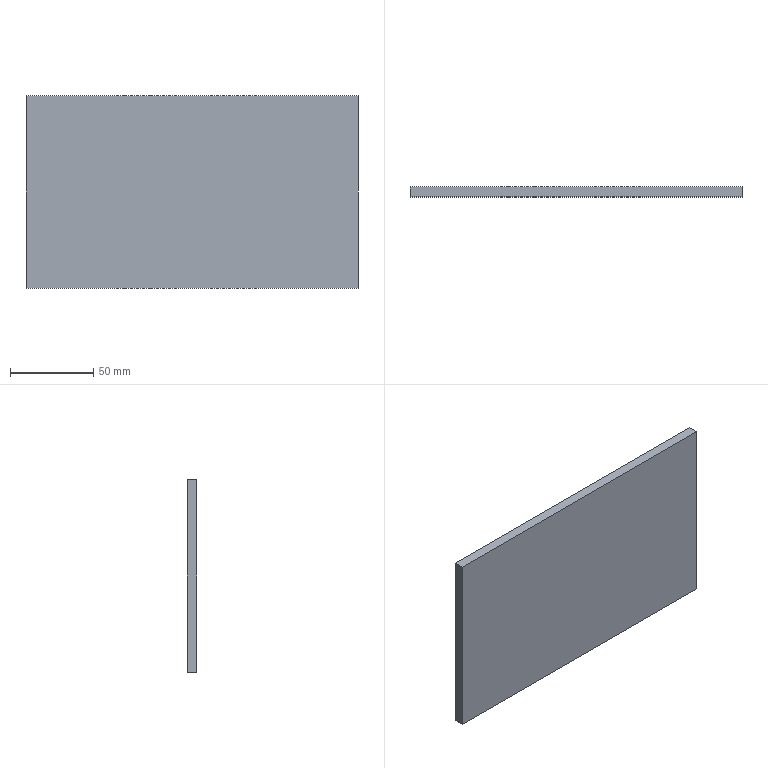Component | SolidWorks | THK-B1013LowerSupportPlate-4 | 1 solid | 6 faces | box 200 x 6 x 116 mm | volume 139200 mm3 | plane 6 | material Q235A
build123d program:
from build123d import *

# Parameters (mm, degrees)
SKETCH1_W           = 200
SKETCH1_H           = 116
BOSS_EXTRUDE1_DEPTH = 3


with BuildPart() as part:
    # Sketch1 → Boss-Extrude1 (new, symmetric)
    with BuildSketch(Plane(origin=(0, 0, 0), x_dir=(1, 0, 0), z_dir=(0, 1, 0))):
        Rectangle(SKETCH1_W, SKETCH1_H)
    extrude(amount=BOSS_EXTRUDE1_DEPTH, both=True)


solid = part.part

# Placed as in the assembly
solid = solid.moved(Location((222, -203, -200), (0, 0, 0)))
STEP:
#1=COLOUR_RGB('',0.7922,0.8196,0.9333);
#2=FILL_AREA_STYLE_COLOUR('',#1);
#3=FILL_AREA_STYLE('',(#2));
#4=SURFACE_STYLE_FILL_AREA(#3);
#5=SURFACE_SIDE_STYLE('',(#4));
#6=SURFACE_STYLE_USAGE(.BOTH.,#5);
#7=PRESENTATION_STYLE_ASSIGNMENT((#6));
#8=CARTESIAN_POINT('',(12.677,-8.11,-5.591));
#9=VERTEX_POINT('',#8);
#10=CARTESIAN_POINT('',(12.677,-8.11,-10.157));
#11=VERTEX_POINT('',#10);
#12=CARTESIAN_POINT('',(12.677,-8.11,-5.591));
#13=DIRECTION('',(0.,0.,-1.));
#14=VECTOR('',#13,39.37);
#15=LINE('',#12,#14);
#16=EDGE_CURVE('',#9,#11,#15,.T.);
#17=ORIENTED_EDGE('',*,*,#16,.T.);
#18=CARTESIAN_POINT('',(12.677,-7.874,-10.157));
#19=VERTEX_POINT('',#18);
#20=CARTESIAN_POINT('',(12.677,-7.874,-10.157));
#21=DIRECTION('',(0.,-1.,0.));
#22=VECTOR('',#21,39.37);
#23=LINE('',#20,#22);
#24=EDGE_CURVE('',#19,#11,#23,.T.);
#25=ORIENTED_EDGE('',*,*,#24,.F.);
#26=CARTESIAN_POINT('',(12.677,-7.874,-5.591));
#27=VERTEX_POINT('',#26);
#28=CARTESIAN_POINT('',(12.677,-7.874,-5.591));
#29=DIRECTION('',(0.,0.,-1.));
#30=VECTOR('',#29,39.37);
#31=LINE('',#28,#30);
#32=EDGE_CURVE('',#27,#19,#31,.T.);
#33=ORIENTED_EDGE('',*,*,#32,.F.);
#34=CARTESIAN_POINT('',(12.677,-7.874,-5.591));
#35=DIRECTION('',(0.,-1.,0.));
#36=VECTOR('',#35,39.37);
#37=LINE('',#34,#36);
#38=EDGE_CURVE('',#27,#9,#37,.T.);
#39=ORIENTED_EDGE('',*,*,#38,.T.);
#40=EDGE_LOOP('',(#17,#25,#33,#39));
#41=FACE_OUTER_BOUND('',#40,.T.);
#42=CARTESIAN_POINT('',(12.677,-7.874,-5.591));
#43=DIRECTION('',(-1.,0.,0.));
#44=DIRECTION('',(0.,0.,1.));
#45=AXIS2_PLACEMENT_3D('',#42,#43,#44);
#46=PLANE('',#45);
#47=ADVANCED_FACE('',(#41),#46,.F.);
#48=CARTESIAN_POINT('',(4.803,-8.11,-10.157));
#49=VERTEX_POINT('',#48);
#50=CARTESIAN_POINT('',(4.803,-8.11,-10.157));
#51=DIRECTION('',(-1.,0.,0.));
#52=VECTOR('',#51,39.37);
#53=LINE('',#50,#52);
#54=EDGE_CURVE('',#11,#49,#53,.T.);
#55=ORIENTED_EDGE('',*,*,#54,.T.);
#56=CARTESIAN_POINT('',(4.803,-7.874,-10.157));
#57=VERTEX_POINT('',#56);
#58=CARTESIAN_POINT('',(4.803,-7.874,-10.157));
#59=DIRECTION('',(0.,-1.,0.));
#60=VECTOR('',#59,39.37);
#61=LINE('',#58,#60);
#62=EDGE_CURVE('',#57,#49,#61,.T.);
#63=ORIENTED_EDGE('',*,*,#62,.F.);
#64=CARTESIAN_POINT('',(4.803,-7.874,-10.157));
#65=DIRECTION('',(-1.,0.,0.));
#66=VECTOR('',#65,39.37);
#67=LINE('',#64,#66);
#68=EDGE_CURVE('',#19,#57,#67,.T.);
#69=ORIENTED_EDGE('',*,*,#68,.F.);
#70=ORIENTED_EDGE('',*,*,#24,.T.);
#71=EDGE_LOOP('',(#55,#63,#69,#70));
#72=FACE_OUTER_BOUND('',#71,.T.);
#73=CARTESIAN_POINT('',(4.803,-7.874,-10.157));
#74=DIRECTION('',(0.,0.,1.));
#75=DIRECTION('',(1.,0.,0.));
#76=AXIS2_PLACEMENT_3D('',#73,#74,#75);
#77=PLANE('',#76);
#78=ADVANCED_FACE('',(#72),#77,.F.);
#79=CARTESIAN_POINT('',(4.803,-8.11,-5.591));
#80=VERTEX_POINT('',#79);
#81=CARTESIAN_POINT('',(4.803,-8.11,-5.591));
#82=DIRECTION('',(0.,0.,1.));
#83=VECTOR('',#82,39.37);
#84=LINE('',#81,#83);
#85=EDGE_CURVE('',#49,#80,#84,.T.);
#86=ORIENTED_EDGE('',*,*,#85,.T.);
#87=CARTESIAN_POINT('',(4.803,-7.874,-5.591));
#88=VERTEX_POINT('',#87);
#89=CARTESIAN_POINT('',(4.803,-7.874,-5.591));
#90=DIRECTION('',(0.,-1.,0.));
#91=VECTOR('',#90,39.37);
#92=LINE('',#89,#91);
#93=EDGE_CURVE('',#88,#80,#92,.T.);
#94=ORIENTED_EDGE('',*,*,#93,.F.);
#95=CARTESIAN_POINT('',(4.803,-7.874,-5.591));
#96=DIRECTION('',(0.,0.,1.));
#97=VECTOR('',#96,39.37);
#98=LINE('',#95,#97);
#99=EDGE_CURVE('',#57,#88,#98,.T.);
#100=ORIENTED_EDGE('',*,*,#99,.F.);
#101=ORIENTED_EDGE('',*,*,#62,.T.);
#102=EDGE_LOOP('',(#86,#94,#100,#101));
#103=FACE_OUTER_BOUND('',#102,.T.);
#104=CARTESIAN_POINT('',(4.803,-7.874,-5.591));
#105=DIRECTION('',(1.,0.,0.));
#106=DIRECTION('',(0.,0.,-1.));
#107=AXIS2_PLACEMENT_3D('',#104,#105,#106);
#108=PLANE('',#107);
#109=ADVANCED_FACE('',(#103),#108,.F.);
#110=CARTESIAN_POINT('',(4.803,-8.11,-5.591));
#111=DIRECTION('',(1.,0.,0.));
#112=VECTOR('',#111,39.37);
#113=LINE('',#110,#112);
#114=EDGE_CURVE('',#80,#9,#113,.T.);
#115=ORIENTED_EDGE('',*,*,#114,.T.);
#116=ORIENTED_EDGE('',*,*,#38,.F.);
#117=CARTESIAN_POINT('',(4.803,-7.874,-5.591));
#118=DIRECTION('',(1.,0.,0.));
#119=VECTOR('',#118,39.37);
#120=LINE('',#117,#119);
#121=EDGE_CURVE('',#88,#27,#120,.T.);
#122=ORIENTED_EDGE('',*,*,#121,.F.);
#123=ORIENTED_EDGE('',*,*,#93,.T.);
#124=EDGE_LOOP('',(#115,#116,#122,#123));
#125=FACE_OUTER_BOUND('',#124,.T.);
#126=CARTESIAN_POINT('',(4.803,-7.874,-5.591));
#127=DIRECTION('',(0.,0.,-1.));
#128=DIRECTION('',(-1.,0.,0.));
#129=AXIS2_PLACEMENT_3D('',#126,#127,#128);
#130=PLANE('',#129);
#131=ADVANCED_FACE('',(#125),#130,.F.);
#132=ORIENTED_EDGE('',*,*,#32,.T.);
#133=ORIENTED_EDGE('',*,*,#68,.T.);
#134=ORIENTED_EDGE('',*,*,#99,.T.);
#135=ORIENTED_EDGE('',*,*,#121,.T.);
#136=EDGE_LOOP('',(#132,#133,#134,#135));
#137=FACE_OUTER_BOUND('',#136,.T.);
#138=CARTESIAN_POINT('',(8.74,-7.874,-7.874));
#139=DIRECTION('',(0.,-1.,0.));
#140=DIRECTION('',(0.,0.,-1.));
#141=AXIS2_PLACEMENT_3D('',#138,#139,#140);
#142=PLANE('',#141);
#143=ADVANCED_FACE('',(#137),#142,.F.);
#144=ORIENTED_EDGE('',*,*,#16,.F.);
#145=ORIENTED_EDGE('',*,*,#114,.F.);
#146=ORIENTED_EDGE('',*,*,#85,.F.);
#147=ORIENTED_EDGE('',*,*,#54,.F.);
#148=EDGE_LOOP('',(#144,#145,#146,#147));
#149=FACE_OUTER_BOUND('',#148,.T.);
#150=CARTESIAN_POINT('',(8.74,-8.11,-7.874));
#151=DIRECTION('',(0.,-1.,0.));
#152=DIRECTION('',(0.,0.,-1.));
#153=AXIS2_PLACEMENT_3D('',#150,#151,#152);
#154=PLANE('',#153);
#155=ADVANCED_FACE('',(#149),#154,.T.);
#156=CLOSED_SHELL('',(#47,#78,#109,#131,#143,#155));
#157=MANIFOLD_SOLID_BREP('',#156);
#158=STYLED_ITEM('',(#7),#157);
#159=PRESENTATION_LAYER_ASSIGNMENT('','',(#158));
#160=CARTESIAN_POINT('',(0.,0.,0.));
#161=DIRECTION('',(0.,0.,1.));
#162=DIRECTION('',(1.,0.,0.));
#163=AXIS2_PLACEMENT_3D('',#160,#161,#162);
#164=(LENGTH_UNIT()NAMED_UNIT(*)SI_UNIT($,.METRE.));
#165=LENGTH_MEASURE_WITH_UNIT(LENGTH_MEASURE(0.0254),#164);
#166=DIMENSIONAL_EXPONENTS(1.,0.,0.,0.,0.,0.,0.);
#167=(CONVERSION_BASED_UNIT('',#165)LENGTH_UNIT()NAMED_UNIT(#166));
#168=UNCERTAINTY_MEASURE_WITH_UNIT(LENGTH_MEASURE(0.00001),#167,'','');
#169=(NAMED_UNIT(*)PLANE_ANGLE_UNIT()SI_UNIT($,.RADIAN.));
#170=(NAMED_UNIT(*)SI_UNIT($,.STERADIAN.)SOLID_ANGLE_UNIT());
#171=(GEOMETRIC_REPRESENTATION_CONTEXT(3)GLOBAL_UNCERTAINTY_ASSIGNED_CONTEXT((#168))GLOBAL_UNIT_ASSIGNED_CONTEXT((#167,#169,#170))REPRESENTATION_CONTEXT('',''));
#172=ADVANCED_BREP_SHAPE_REPRESENTATION('',(#157,#163),#171);
#173=(LENGTH_UNIT()NAMED_UNIT(*)SI_UNIT($,.METRE.));
#174=LENGTH_MEASURE_WITH_UNIT(LENGTH_MEASURE(0.0254),#173);
#175=DIMENSIONAL_EXPONENTS(1.,0.,0.,0.,0.,0.,0.);
#176=(CONVERSION_BASED_UNIT('',#174)LENGTH_UNIT()NAMED_UNIT(#175));
#177=UNCERTAINTY_MEASURE_WITH_UNIT(LENGTH_MEASURE(0.00001),#176,'','');
#178=(NAMED_UNIT(*)PLANE_ANGLE_UNIT()SI_UNIT($,.RADIAN.));
#179=(NAMED_UNIT(*)SI_UNIT($,.STERADIAN.)SOLID_ANGLE_UNIT());
#180=(GEOMETRIC_REPRESENTATION_CONTEXT(3)GLOBAL_UNCERTAINTY_ASSIGNED_CONTEXT((#177))GLOBAL_UNIT_ASSIGNED_CONTEXT((#176,#178,#179))REPRESENTATION_CONTEXT('',''));
#181=MECHANICAL_DESIGN_GEOMETRIC_PRESENTATION_REPRESENTATION('',(#158),#180);